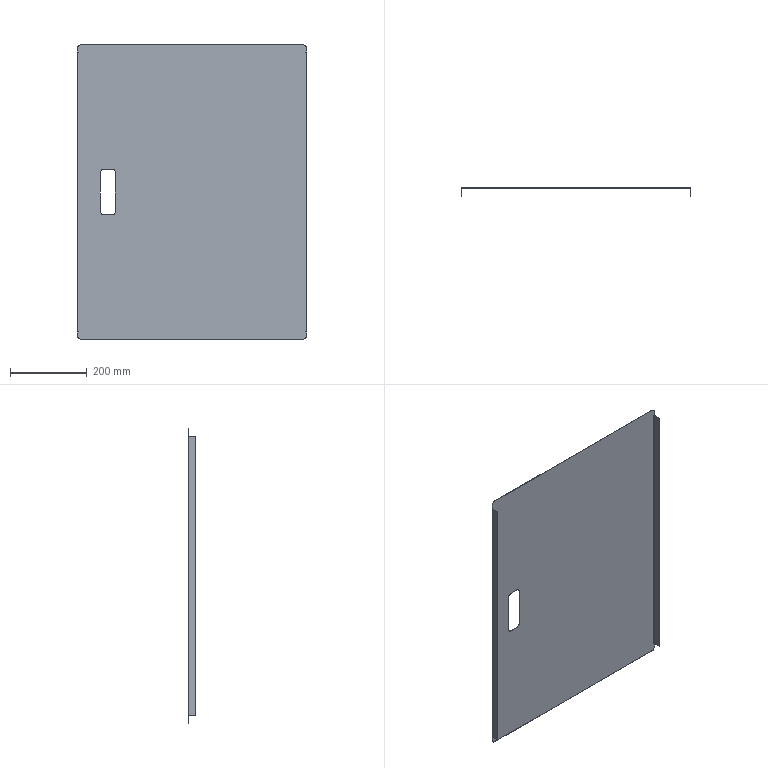Component | SolidWorks | DoorPlate-1_OuterDoorPanel-1 | 1 solid | 50 faces | volume 388415 mm3 | plane 38 | cylinder 12 | commonest cylinder face diameters 20 x8 3.6 x2 2 x2 | material 304